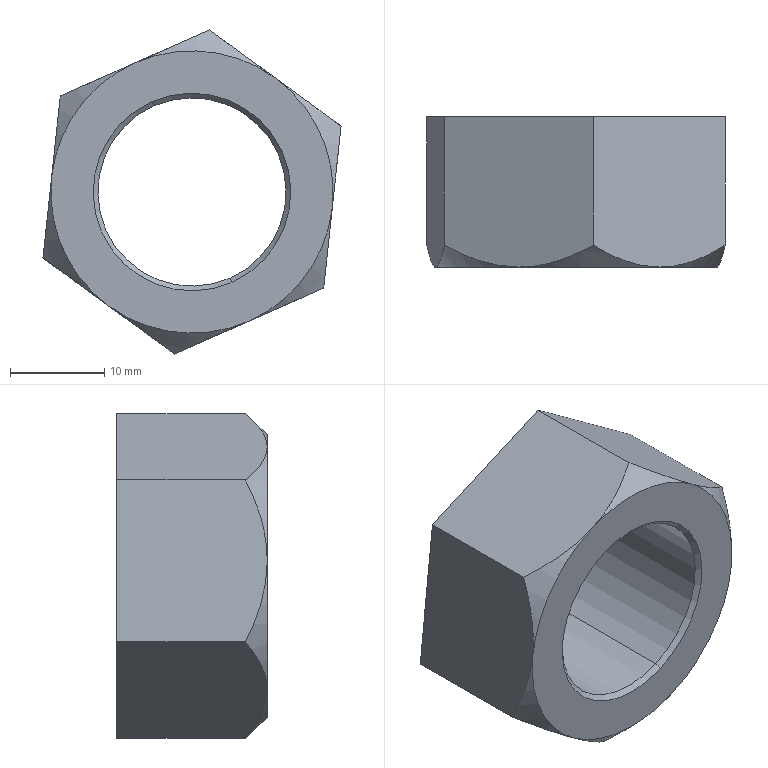Component | SolidWorks | 30-01A-1_Wheel-322-1_FBR100-20-322-1_FBR20nut-322-1 | 1 solid | 20 faces | box 31.68 x 16 x 34.44 mm | volume 7377 mm3 | cone 10 | plane 8 | cylinder 2 | commonest cylinder face diameters 20 x2
STEP:
#1=CARTESIAN_POINT('',(9.316,-22.179,-1.147));
#2=VERTEX_POINT('',#1);
#3=CARTESIAN_POINT('',(8.997,-22.179,-0.4274));
#4=VERTEX_POINT('',#3);
#5=CARTESIAN_POINT('',(9.156,-22.179,-0.7874));
#6=DIRECTION('',(-0.,-1.,0.));
#7=DIRECTION('',(-0.4048,0.,0.9144));
#8=AXIS2_PLACEMENT_3D('',#5,#6,#7);
#9=CIRCLE('',#8,0.3937);
#10=EDGE_CURVE('',#2,#4,#9,.T.);
#11=ORIENTED_EDGE('',*,*,#10,.T.);
#12=CARTESIAN_POINT('',(8.989,-22.159,-0.4094));
#13=VERTEX_POINT('',#12);
#14=CARTESIAN_POINT('',(8.989,-22.159,-0.4094));
#15=DIRECTION('',(-0.2863,0.7071,0.6466));
#16=VECTOR('',#15,39.37);
#17=LINE('',#14,#16);
#18=EDGE_CURVE('',#4,#13,#17,.T.);
#19=ORIENTED_EDGE('',*,*,#18,.T.);
#20=CARTESIAN_POINT('',(9.324,-22.159,-1.165));
#21=VERTEX_POINT('',#20);
#22=CARTESIAN_POINT('',(9.156,-22.159,-0.7874));
#23=DIRECTION('',(-0.,-1.,0.));
#24=DIRECTION('',(-0.4048,0.,0.9144));
#25=AXIS2_PLACEMENT_3D('',#22,#23,#24);
#26=CIRCLE('',#25,0.4134);
#27=EDGE_CURVE('',#21,#13,#26,.T.);
#28=ORIENTED_EDGE('',*,*,#27,.F.);
#29=CARTESIAN_POINT('',(9.324,-22.159,-1.165));
#30=DIRECTION('',(0.2863,0.7071,-0.6466));
#31=VECTOR('',#30,39.37);
#32=LINE('',#29,#31);
#33=EDGE_CURVE('',#2,#21,#32,.T.);
#34=ORIENTED_EDGE('',*,*,#33,.F.);
#35=EDGE_LOOP('',(#11,#19,#28,#34));
#36=FACE_OUTER_BOUND('',#35,.T.);
#37=CARTESIAN_POINT('',(9.156,-22.159,-0.7874));
#38=DIRECTION('',(0.,1.,-0.));
#39=DIRECTION('',(0.4048,0.,-0.9144));
#40=AXIS2_PLACEMENT_3D('',#37,#38,#39);
#41=CONICAL_SURFACE('',#40,0.4134,0.7854);
#42=ADVANCED_FACE('',(#36),#41,.F.);
#43=ORIENTED_EDGE('',*,*,#10,.F.);
#44=CARTESIAN_POINT('',(9.316,-22.769,-1.147));
#45=VERTEX_POINT('',#44);
#46=CARTESIAN_POINT('',(9.316,-22.159,-1.147));
#47=DIRECTION('',(-0.,-1.,0.));
#48=VECTOR('',#47,39.37);
#49=LINE('',#46,#48);
#50=EDGE_CURVE('',#2,#45,#49,.T.);
#51=ORIENTED_EDGE('',*,*,#50,.T.);
#52=CARTESIAN_POINT('',(8.997,-22.769,-0.4274));
#53=VERTEX_POINT('',#52);
#54=CARTESIAN_POINT('',(9.156,-22.769,-0.7874));
#55=DIRECTION('',(-0.,-1.,0.));
#56=DIRECTION('',(-0.4048,0.,0.9144));
#57=AXIS2_PLACEMENT_3D('',#54,#55,#56);
#58=CIRCLE('',#57,0.3937);
#59=EDGE_CURVE('',#45,#53,#58,.T.);
#60=ORIENTED_EDGE('',*,*,#59,.T.);
#61=CARTESIAN_POINT('',(8.997,-22.159,-0.4274));
#62=DIRECTION('',(-0.,-1.,0.));
#63=VECTOR('',#62,39.37);
#64=LINE('',#61,#63);
#65=EDGE_CURVE('',#4,#53,#64,.T.);
#66=ORIENTED_EDGE('',*,*,#65,.F.);
#67=EDGE_LOOP('',(#43,#51,#60,#66));
#68=FACE_OUTER_BOUND('',#67,.T.);
#69=CARTESIAN_POINT('',(9.156,-22.159,-0.7874));
#70=DIRECTION('',(-0.,-1.,0.));
#71=DIRECTION('',(-0.4048,0.,0.9144));
#72=AXIS2_PLACEMENT_3D('',#69,#70,#71);
#73=CYLINDRICAL_SURFACE('',#72,0.3937);
#74=ADVANCED_FACE('',(#68),#73,.F.);
#75=ORIENTED_EDGE('',*,*,#59,.F.);
#76=CARTESIAN_POINT('',(9.324,-22.789,-1.165));
#77=VERTEX_POINT('',#76);
#78=CARTESIAN_POINT('',(9.316,-22.769,-1.147));
#79=DIRECTION('',(0.2863,-0.7071,-0.6466));
#80=VECTOR('',#79,39.37);
#81=LINE('',#78,#80);
#82=EDGE_CURVE('',#45,#77,#81,.T.);
#83=ORIENTED_EDGE('',*,*,#82,.T.);
#84=CARTESIAN_POINT('',(8.989,-22.789,-0.4094));
#85=VERTEX_POINT('',#84);
#86=CARTESIAN_POINT('',(9.156,-22.789,-0.7874));
#87=DIRECTION('',(-0.,-1.,0.));
#88=DIRECTION('',(-0.4048,0.,0.9144));
#89=AXIS2_PLACEMENT_3D('',#86,#87,#88);
#90=CIRCLE('',#89,0.4134);
#91=EDGE_CURVE('',#77,#85,#90,.T.);
#92=ORIENTED_EDGE('',*,*,#91,.T.);
#93=CARTESIAN_POINT('',(8.997,-22.769,-0.4274));
#94=DIRECTION('',(-0.2863,-0.7071,0.6466));
#95=VECTOR('',#94,39.37);
#96=LINE('',#93,#95);
#97=EDGE_CURVE('',#53,#85,#96,.T.);
#98=ORIENTED_EDGE('',*,*,#97,.F.);
#99=EDGE_LOOP('',(#75,#83,#92,#98));
#100=FACE_OUTER_BOUND('',#99,.T.);
#101=CARTESIAN_POINT('',(9.156,-22.769,-0.7874));
#102=DIRECTION('',(-0.,-1.,0.));
#103=DIRECTION('',(-0.4048,0.,0.9144));
#104=AXIS2_PLACEMENT_3D('',#101,#102,#103);
#105=CONICAL_SURFACE('',#104,0.3937,0.7854);
#106=ADVANCED_FACE('',(#100),#105,.F.);
#107=CARTESIAN_POINT('',(8.917,-22.789,-0.2474));
#108=VERTEX_POINT('',#107);
#109=CARTESIAN_POINT('',(8.569,-22.789,-0.7245));
#110=VERTEX_POINT('',#109);
#111=CARTESIAN_POINT('',(9.156,-22.789,-0.7874));
#112=DIRECTION('',(-0.,-1.,0.));
#113=DIRECTION('',(-0.4048,0.,0.9144));
#114=AXIS2_PLACEMENT_3D('',#111,#112,#113);
#115=CIRCLE('',#114,0.5906);
#116=EDGE_CURVE('',#108,#110,#115,.T.);
#117=ORIENTED_EDGE('',*,*,#116,.T.);
#118=CARTESIAN_POINT('',(8.808,-22.789,-1.264));
#119=VERTEX_POINT('',#118);
#120=CARTESIAN_POINT('',(9.156,-22.789,-0.7874));
#121=DIRECTION('',(-0.,-1.,0.));
#122=DIRECTION('',(-0.4048,0.,0.9144));
#123=AXIS2_PLACEMENT_3D('',#120,#121,#122);
#124=CIRCLE('',#123,0.5906);
#125=EDGE_CURVE('',#110,#119,#124,.T.);
#126=ORIENTED_EDGE('',*,*,#125,.T.);
#127=CARTESIAN_POINT('',(9.395,-22.789,-1.327));
#128=VERTEX_POINT('',#127);
#129=CARTESIAN_POINT('',(9.156,-22.789,-0.7874));
#130=DIRECTION('',(-0.,-1.,0.));
#131=DIRECTION('',(-0.4048,0.,0.9144));
#132=AXIS2_PLACEMENT_3D('',#129,#130,#131);
#133=CIRCLE('',#132,0.5906);
#134=EDGE_CURVE('',#119,#128,#133,.T.);
#135=ORIENTED_EDGE('',*,*,#134,.T.);
#136=CARTESIAN_POINT('',(9.743,-22.789,-0.8503));
#137=VERTEX_POINT('',#136);
#138=CARTESIAN_POINT('',(9.156,-22.789,-0.7874));
#139=DIRECTION('',(-0.,-1.,0.));
#140=DIRECTION('',(-0.4048,0.,0.9144));
#141=AXIS2_PLACEMENT_3D('',#138,#139,#140);
#142=CIRCLE('',#141,0.5906);
#143=EDGE_CURVE('',#128,#137,#142,.T.);
#144=ORIENTED_EDGE('',*,*,#143,.T.);
#145=CARTESIAN_POINT('',(9.504,-22.789,-0.3104));
#146=VERTEX_POINT('',#145);
#147=CARTESIAN_POINT('',(9.156,-22.789,-0.7874));
#148=DIRECTION('',(-0.,-1.,0.));
#149=DIRECTION('',(-0.4048,0.,0.9144));
#150=AXIS2_PLACEMENT_3D('',#147,#148,#149);
#151=CIRCLE('',#150,0.5906);
#152=EDGE_CURVE('',#137,#146,#151,.T.);
#153=ORIENTED_EDGE('',*,*,#152,.T.);
#154=CARTESIAN_POINT('',(9.156,-22.789,-0.7874));
#155=DIRECTION('',(-0.,-1.,0.));
#156=DIRECTION('',(-0.4048,0.,0.9144));
#157=AXIS2_PLACEMENT_3D('',#154,#155,#156);
#158=CIRCLE('',#157,0.5906);
#159=EDGE_CURVE('',#146,#108,#158,.T.);
#160=ORIENTED_EDGE('',*,*,#159,.T.);
#161=EDGE_LOOP('',(#117,#126,#135,#144,#153,#160));
#162=FACE_OUTER_BOUND('',#161,.T.);
#163=CARTESIAN_POINT('',(9.156,-22.789,-0.7874));
#164=DIRECTION('',(-0.,-1.,0.));
#165=DIRECTION('',(-0.4048,0.,0.9144));
#166=AXIS2_PLACEMENT_3D('',#163,#164,#165);
#167=CIRCLE('',#166,0.4134);
#168=EDGE_CURVE('',#85,#77,#167,.T.);
#169=ORIENTED_EDGE('',*,*,#168,.F.);
#170=ORIENTED_EDGE('',*,*,#91,.F.);
#171=EDGE_LOOP('',(#169,#170));
#172=FACE_BOUND('',#171,.T.);
#173=CARTESIAN_POINT('',(9.156,-22.789,-0.7874));
#174=DIRECTION('',(0.,1.,-0.));
#175=DIRECTION('',(0.4048,-0.,-0.9144));
#176=AXIS2_PLACEMENT_3D('',#173,#174,#175);
#177=PLANE('',#176);
#178=ADVANCED_FACE('',(#162,#172),#177,.F.);
#179=CARTESIAN_POINT('',(9.78,-22.159,-0.5113));
#180=VERTEX_POINT('',#179);
#181=CARTESIAN_POINT('',(9.229,-22.159,-0.1094));
#182=VERTEX_POINT('',#181);
#183=CARTESIAN_POINT('',(9.78,-22.159,-0.5113));
#184=DIRECTION('',(-0.8078,0.,0.5895));
#185=VECTOR('',#184,39.37);
#186=LINE('',#183,#185);
#187=EDGE_CURVE('',#180,#182,#186,.T.);
#188=ORIENTED_EDGE('',*,*,#187,.F.);
#189=CARTESIAN_POINT('',(9.707,-22.159,-1.189));
#190=VERTEX_POINT('',#189);
#191=CARTESIAN_POINT('',(9.707,-22.159,-1.189));
#192=DIRECTION('',(0.1066,0.,0.9943));
#193=VECTOR('',#192,39.37);
#194=LINE('',#191,#193);
#195=EDGE_CURVE('',#190,#180,#194,.T.);
#196=ORIENTED_EDGE('',*,*,#195,.F.);
#197=CARTESIAN_POINT('',(9.084,-22.159,-1.465));
#198=VERTEX_POINT('',#197);
#199=CARTESIAN_POINT('',(9.084,-22.159,-1.465));
#200=DIRECTION('',(0.9144,-0.,0.4048));
#201=VECTOR('',#200,39.37);
#202=LINE('',#199,#201);
#203=EDGE_CURVE('',#198,#190,#202,.T.);
#204=ORIENTED_EDGE('',*,*,#203,.F.);
#205=CARTESIAN_POINT('',(8.533,-22.159,-1.063));
#206=VERTEX_POINT('',#205);
#207=CARTESIAN_POINT('',(8.533,-22.159,-1.063));
#208=DIRECTION('',(0.8078,-0.,-0.5895));
#209=VECTOR('',#208,39.37);
#210=LINE('',#207,#209);
#211=EDGE_CURVE('',#206,#198,#210,.T.);
#212=ORIENTED_EDGE('',*,*,#211,.F.);
#213=CARTESIAN_POINT('',(8.605,-22.159,-0.3854));
#214=VERTEX_POINT('',#213);
#215=CARTESIAN_POINT('',(8.605,-22.159,-0.3854));
#216=DIRECTION('',(-0.1066,-0.,-0.9943));
#217=VECTOR('',#216,39.37);
#218=LINE('',#215,#217);
#219=EDGE_CURVE('',#214,#206,#218,.T.);
#220=ORIENTED_EDGE('',*,*,#219,.F.);
#221=CARTESIAN_POINT('',(9.229,-22.159,-0.1094));
#222=DIRECTION('',(-0.9144,0.,-0.4048));
#223=VECTOR('',#222,39.37);
#224=LINE('',#221,#223);
#225=EDGE_CURVE('',#182,#214,#224,.T.);
#226=ORIENTED_EDGE('',*,*,#225,.F.);
#227=EDGE_LOOP('',(#188,#196,#204,#212,#220,#226));
#228=FACE_OUTER_BOUND('',#227,.T.);
#229=ORIENTED_EDGE('',*,*,#27,.T.);
#230=CARTESIAN_POINT('',(9.156,-22.159,-0.7874));
#231=DIRECTION('',(-0.,-1.,0.));
#232=DIRECTION('',(-0.4048,0.,0.9144));
#233=AXIS2_PLACEMENT_3D('',#230,#231,#232);
#234=CIRCLE('',#233,0.4134);
#235=EDGE_CURVE('',#13,#21,#234,.T.);
#236=ORIENTED_EDGE('',*,*,#235,.T.);
#237=EDGE_LOOP('',(#229,#236));
#238=FACE_BOUND('',#237,.T.);
#239=CARTESIAN_POINT('',(8.508,-22.159,-1.074));
#240=DIRECTION('',(-0.,-1.,0.));
#241=DIRECTION('',(-0.4048,0.,0.9144));
#242=AXIS2_PLACEMENT_3D('',#239,#240,#241);
#243=PLANE('',#242);
#244=ADVANCED_FACE('',(#228,#238),#243,.F.);
#245=CARTESIAN_POINT('',(9.707,-22.698,-1.189));
#246=VERTEX_POINT('',#245);
#247=CARTESIAN_POINT('',(9.395,-22.789,-1.327));
#248=CARTESIAN_POINT('',(9.409,-22.789,-1.321));
#249=CARTESIAN_POINT('',(9.423,-22.789,-1.315));
#250=CARTESIAN_POINT('',(9.45,-22.786,-1.303));
#251=CARTESIAN_POINT('',(9.463,-22.785,-1.297));
#252=CARTESIAN_POINT('',(9.504,-22.778,-1.279));
#253=CARTESIAN_POINT('',(9.53,-22.772,-1.268));
#254=CARTESIAN_POINT('',(9.582,-22.756,-1.245));
#255=CARTESIAN_POINT('',(9.608,-22.746,-1.233));
#256=CARTESIAN_POINT('',(9.658,-22.723,-1.211));
#257=CARTESIAN_POINT('',(9.683,-22.711,-1.2));
#258=CARTESIAN_POINT('',(9.707,-22.698,-1.189));
#259=B_SPLINE_CURVE_WITH_KNOTS('',3,(#247,#248,#249,#250,#251,#252,#253,#254,#255,#256,#257,#258),.UNSPECIFIED.,.F.,.F.,(4,2,2,2,2,4),(0.01814,0.01926,0.02038,0.02262,0.02486,0.02711),.UNSPECIFIED.);
#260=EDGE_CURVE('',#128,#246,#259,.T.);
#261=ORIENTED_EDGE('',*,*,#260,.T.);
#262=CARTESIAN_POINT('',(9.707,-22.698,-1.189));
#263=CARTESIAN_POINT('',(9.713,-22.725,-1.136));
#264=CARTESIAN_POINT('',(9.719,-22.747,-1.082));
#265=CARTESIAN_POINT('',(9.728,-22.772,-0.9974));
#266=CARTESIAN_POINT('',(9.731,-22.778,-0.9687));
#267=CARTESIAN_POINT('',(9.737,-22.787,-0.9102));
#268=CARTESIAN_POINT('',(9.74,-22.789,-0.88));
#269=CARTESIAN_POINT('',(9.743,-22.789,-0.8503));
#270=B_SPLINE_CURVE_WITH_KNOTS('',3,(#262,#263,#264,#265,#266,#267,#268,#269),.UNSPECIFIED.,.F.,.F.,(4,2,2,4),(0.00000025,0.004489,0.006733,0.008977),.UNSPECIFIED.);
#271=EDGE_CURVE('',#246,#137,#270,.T.);
#272=ORIENTED_EDGE('',*,*,#271,.T.);
#273=ORIENTED_EDGE('',*,*,#143,.F.);
#274=EDGE_LOOP('',(#261,#272,#273));
#275=FACE_OUTER_BOUND('',#274,.T.);
#276=CARTESIAN_POINT('',(9.156,-22.671,-0.7874));
#277=DIRECTION('',(0.,1.,-0.));
#278=DIRECTION('',(0.4048,0.,-0.9144));
#279=AXIS2_PLACEMENT_3D('',#276,#277,#278);
#280=CONICAL_SURFACE('',#279,0.7087,0.7854);
#281=ADVANCED_FACE('',(#275),#280,.T.);
#282=ORIENTED_EDGE('',*,*,#152,.F.);
#283=CARTESIAN_POINT('',(9.78,-22.698,-0.5113));
#284=VERTEX_POINT('',#283);
#285=CARTESIAN_POINT('',(9.743,-22.789,-0.8503));
#286=CARTESIAN_POINT('',(9.75,-22.789,-0.7914));
#287=CARTESIAN_POINT('',(9.756,-22.78,-0.7334));
#288=CARTESIAN_POINT('',(9.768,-22.747,-0.6191));
#289=CARTESIAN_POINT('',(9.774,-22.724,-0.5644));
#290=CARTESIAN_POINT('',(9.78,-22.698,-0.5113));
#291=B_SPLINE_CURVE_WITH_KNOTS('',3,(#285,#286,#287,#288,#289,#290),.UNSPECIFIED.,.F.,.F.,(4,2,4),(0.008977,0.01343,0.01789),.UNSPECIFIED.);
#292=EDGE_CURVE('',#137,#284,#291,.T.);
#293=ORIENTED_EDGE('',*,*,#292,.T.);
#294=CARTESIAN_POINT('',(9.78,-22.698,-0.5113));
#295=CARTESIAN_POINT('',(9.737,-22.725,-0.4798));
#296=CARTESIAN_POINT('',(9.692,-22.747,-0.4476));
#297=CARTESIAN_POINT('',(9.624,-22.772,-0.3975));
#298=CARTESIAN_POINT('',(9.601,-22.778,-0.3805));
#299=CARTESIAN_POINT('',(9.553,-22.787,-0.3458));
#300=CARTESIAN_POINT('',(9.529,-22.789,-0.328));
#301=CARTESIAN_POINT('',(9.504,-22.789,-0.3104));
#302=B_SPLINE_CURVE_WITH_KNOTS('',3,(#294,#295,#296,#297,#298,#299,#300,#301),.UNSPECIFIED.,.F.,.F.,(4,2,2,4),(0.00000025,0.004489,0.006733,0.008977),.UNSPECIFIED.);
#303=EDGE_CURVE('',#284,#146,#302,.T.);
#304=ORIENTED_EDGE('',*,*,#303,.T.);
#305=EDGE_LOOP('',(#282,#293,#304));
#306=FACE_OUTER_BOUND('',#305,.T.);
#307=CARTESIAN_POINT('',(9.156,-22.671,-0.7874));
#308=DIRECTION('',(0.,1.,-0.));
#309=DIRECTION('',(0.4048,0.,-0.9144));
#310=AXIS2_PLACEMENT_3D('',#307,#308,#309);
#311=CONICAL_SURFACE('',#310,0.7087,0.7854);
#312=ADVANCED_FACE('',(#306),#311,.T.);
#313=ORIENTED_EDGE('',*,*,#159,.F.);
#314=CARTESIAN_POINT('',(9.229,-22.698,-0.1094));
#315=VERTEX_POINT('',#314);
#316=CARTESIAN_POINT('',(9.504,-22.789,-0.3104));
#317=CARTESIAN_POINT('',(9.457,-22.789,-0.2754));
#318=CARTESIAN_POINT('',(9.409,-22.78,-0.241));
#319=CARTESIAN_POINT('',(9.317,-22.747,-0.1733));
#320=CARTESIAN_POINT('',(9.272,-22.724,-0.1409));
#321=CARTESIAN_POINT('',(9.229,-22.698,-0.1094));
#322=B_SPLINE_CURVE_WITH_KNOTS('',3,(#316,#317,#318,#319,#320,#321),.UNSPECIFIED.,.F.,.F.,(4,2,4),(0.008977,0.01343,0.01789),.UNSPECIFIED.);
#323=EDGE_CURVE('',#146,#315,#322,.T.);
#324=ORIENTED_EDGE('',*,*,#323,.T.);
#325=CARTESIAN_POINT('',(9.229,-22.698,-0.1094));
#326=CARTESIAN_POINT('',(9.205,-22.711,-0.1201));
#327=CARTESIAN_POINT('',(9.18,-22.723,-0.131));
#328=CARTESIAN_POINT('',(9.129,-22.746,-0.1535));
#329=CARTESIAN_POINT('',(9.104,-22.756,-0.1648));
#330=CARTESIAN_POINT('',(9.052,-22.772,-0.1878));
#331=CARTESIAN_POINT('',(9.025,-22.778,-0.1995));
#332=CARTESIAN_POINT('',(8.985,-22.785,-0.2173));
#333=CARTESIAN_POINT('',(8.972,-22.786,-0.2232));
#334=CARTESIAN_POINT('',(8.945,-22.789,-0.2353));
#335=CARTESIAN_POINT('',(8.931,-22.789,-0.2414));
#336=CARTESIAN_POINT('',(8.917,-22.789,-0.2474));
#337=B_SPLINE_CURVE_WITH_KNOTS('',3,(#325,#326,#327,#328,#329,#330,#331,#332,#333,#334,#335,#336),.UNSPECIFIED.,.F.,.F.,(4,2,2,2,2,4),(0.0116,0.01384,0.01608,0.01833,0.01945,0.02057),.UNSPECIFIED.);
#338=EDGE_CURVE('',#315,#108,#337,.T.);
#339=ORIENTED_EDGE('',*,*,#338,.T.);
#340=EDGE_LOOP('',(#313,#324,#339));
#341=FACE_OUTER_BOUND('',#340,.T.);
#342=CARTESIAN_POINT('',(9.156,-22.671,-0.7874));
#343=DIRECTION('',(0.,1.,-0.));
#344=DIRECTION('',(0.4048,0.,-0.9144));
#345=AXIS2_PLACEMENT_3D('',#342,#343,#344);
#346=CONICAL_SURFACE('',#345,0.7087,0.7854);
#347=ADVANCED_FACE('',(#341),#346,.T.);
#348=ORIENTED_EDGE('',*,*,#116,.F.);
#349=CARTESIAN_POINT('',(8.605,-22.698,-0.3854));
#350=VERTEX_POINT('',#349);
#351=CARTESIAN_POINT('',(8.917,-22.789,-0.2474));
#352=CARTESIAN_POINT('',(8.862,-22.789,-0.2717));
#353=CARTESIAN_POINT('',(8.809,-22.78,-0.2953));
#354=CARTESIAN_POINT('',(8.731,-22.755,-0.33));
#355=CARTESIAN_POINT('',(8.705,-22.746,-0.3415));
#356=CARTESIAN_POINT('',(8.654,-22.723,-0.3639));
#357=CARTESIAN_POINT('',(8.63,-22.711,-0.3748));
#358=CARTESIAN_POINT('',(8.605,-22.698,-0.3854));
#359=B_SPLINE_CURVE_WITH_KNOTS('',3,(#351,#352,#353,#354,#355,#356,#357,#358),.UNSPECIFIED.,.F.,.F.,(4,2,2,4),(0.02057,0.02506,0.02731,0.02956),.UNSPECIFIED.);
#360=EDGE_CURVE('',#108,#350,#359,.T.);
#361=ORIENTED_EDGE('',*,*,#360,.T.);
#362=CARTESIAN_POINT('',(8.605,-22.698,-0.3854));
#363=CARTESIAN_POINT('',(8.6,-22.725,-0.4386));
#364=CARTESIAN_POINT('',(8.594,-22.747,-0.493));
#365=CARTESIAN_POINT('',(8.585,-22.772,-0.5775));
#366=CARTESIAN_POINT('',(8.582,-22.778,-0.6061));
#367=CARTESIAN_POINT('',(8.576,-22.787,-0.6646));
#368=CARTESIAN_POINT('',(8.572,-22.789,-0.6948));
#369=CARTESIAN_POINT('',(8.569,-22.789,-0.7245));
#370=B_SPLINE_CURVE_WITH_KNOTS('',3,(#362,#363,#364,#365,#366,#367,#368,#369),.UNSPECIFIED.,.F.,.F.,(4,2,2,4),(0.00000025,0.004489,0.006733,0.008977),.UNSPECIFIED.);
#371=EDGE_CURVE('',#350,#110,#370,.T.);
#372=ORIENTED_EDGE('',*,*,#371,.T.);
#373=EDGE_LOOP('',(#348,#361,#372));
#374=FACE_OUTER_BOUND('',#373,.T.);
#375=CARTESIAN_POINT('',(9.156,-22.671,-0.7874));
#376=DIRECTION('',(0.,1.,-0.));
#377=DIRECTION('',(0.4048,0.,-0.9144));
#378=AXIS2_PLACEMENT_3D('',#375,#376,#377);
#379=CONICAL_SURFACE('',#378,0.7087,0.7854);
#380=ADVANCED_FACE('',(#374),#379,.T.);
#381=ORIENTED_EDGE('',*,*,#125,.F.);
#382=CARTESIAN_POINT('',(8.533,-22.698,-1.063));
#383=VERTEX_POINT('',#382);
#384=CARTESIAN_POINT('',(8.569,-22.789,-0.7245));
#385=CARTESIAN_POINT('',(8.563,-22.789,-0.7834));
#386=CARTESIAN_POINT('',(8.557,-22.78,-0.8414));
#387=CARTESIAN_POINT('',(8.544,-22.747,-0.9557));
#388=CARTESIAN_POINT('',(8.538,-22.724,-1.01));
#389=CARTESIAN_POINT('',(8.533,-22.698,-1.063));
#390=B_SPLINE_CURVE_WITH_KNOTS('',3,(#384,#385,#386,#387,#388,#389),.UNSPECIFIED.,.F.,.F.,(4,2,4),(0.008977,0.01343,0.01789),.UNSPECIFIED.);
#391=EDGE_CURVE('',#110,#383,#390,.T.);
#392=ORIENTED_EDGE('',*,*,#391,.T.);
#393=CARTESIAN_POINT('',(8.533,-22.698,-1.063));
#394=CARTESIAN_POINT('',(8.576,-22.725,-1.095));
#395=CARTESIAN_POINT('',(8.62,-22.747,-1.127));
#396=CARTESIAN_POINT('',(8.689,-22.772,-1.177));
#397=CARTESIAN_POINT('',(8.712,-22.778,-1.194));
#398=CARTESIAN_POINT('',(8.76,-22.787,-1.229));
#399=CARTESIAN_POINT('',(8.784,-22.789,-1.247));
#400=CARTESIAN_POINT('',(8.808,-22.789,-1.264));
#401=B_SPLINE_CURVE_WITH_KNOTS('',3,(#393,#394,#395,#396,#397,#398,#399,#400),.UNSPECIFIED.,.F.,.F.,(4,2,2,4),(0.00000025,0.004489,0.006733,0.008977),.UNSPECIFIED.);
#402=EDGE_CURVE('',#383,#119,#401,.T.);
#403=ORIENTED_EDGE('',*,*,#402,.T.);
#404=EDGE_LOOP('',(#381,#392,#403));
#405=FACE_OUTER_BOUND('',#404,.T.);
#406=CARTESIAN_POINT('',(9.156,-22.671,-0.7874));
#407=DIRECTION('',(0.,1.,-0.));
#408=DIRECTION('',(0.4048,0.,-0.9144));
#409=AXIS2_PLACEMENT_3D('',#406,#407,#408);
#410=CONICAL_SURFACE('',#409,0.7087,0.7854);
#411=ADVANCED_FACE('',(#405),#410,.T.);
#412=ORIENTED_EDGE('',*,*,#134,.F.);
#413=CARTESIAN_POINT('',(9.084,-22.698,-1.465));
#414=VERTEX_POINT('',#413);
#415=CARTESIAN_POINT('',(8.808,-22.789,-1.264));
#416=CARTESIAN_POINT('',(8.856,-22.789,-1.299));
#417=CARTESIAN_POINT('',(8.903,-22.78,-1.334));
#418=CARTESIAN_POINT('',(8.996,-22.747,-1.402));
#419=CARTESIAN_POINT('',(9.04,-22.724,-1.434));
#420=CARTESIAN_POINT('',(9.084,-22.698,-1.465));
#421=B_SPLINE_CURVE_WITH_KNOTS('',3,(#415,#416,#417,#418,#419,#420),.UNSPECIFIED.,.F.,.F.,(4,2,4),(0.008977,0.01343,0.01789),.UNSPECIFIED.);
#422=EDGE_CURVE('',#119,#414,#421,.T.);
#423=ORIENTED_EDGE('',*,*,#422,.T.);
#424=CARTESIAN_POINT('',(9.084,-22.698,-1.465));
#425=CARTESIAN_POINT('',(9.108,-22.711,-1.455));
#426=CARTESIAN_POINT('',(9.132,-22.723,-1.444));
#427=CARTESIAN_POINT('',(9.183,-22.746,-1.422));
#428=CARTESIAN_POINT('',(9.209,-22.755,-1.41));
#429=CARTESIAN_POINT('',(9.287,-22.78,-1.375));
#430=CARTESIAN_POINT('',(9.341,-22.789,-1.352));
#431=CARTESIAN_POINT('',(9.395,-22.789,-1.327));
#432=B_SPLINE_CURVE_WITH_KNOTS('',3,(#424,#425,#426,#427,#428,#429,#430,#431),.UNSPECIFIED.,.F.,.F.,(4,2,2,4),(0.00916,0.0114,0.01365,0.01814),.UNSPECIFIED.);
#433=EDGE_CURVE('',#414,#128,#432,.T.);
#434=ORIENTED_EDGE('',*,*,#433,.T.);
#435=EDGE_LOOP('',(#412,#423,#434));
#436=FACE_OUTER_BOUND('',#435,.T.);
#437=CARTESIAN_POINT('',(9.156,-22.671,-0.7874));
#438=DIRECTION('',(0.,1.,-0.));
#439=DIRECTION('',(0.4048,0.,-0.9144));
#440=AXIS2_PLACEMENT_3D('',#437,#438,#439);
#441=CONICAL_SURFACE('',#440,0.7087,0.7854);
#442=ADVANCED_FACE('',(#436),#441,.T.);
#443=CARTESIAN_POINT('',(9.707,-22.829,-1.189));
#444=DIRECTION('',(0.,1.,-0.));
#445=VECTOR('',#444,39.37);
#446=LINE('',#443,#445);
#447=EDGE_CURVE('',#246,#190,#446,.T.);
#448=ORIENTED_EDGE('',*,*,#447,.T.);
#449=ORIENTED_EDGE('',*,*,#195,.T.);
#450=CARTESIAN_POINT('',(9.78,-22.829,-0.5113));
#451=DIRECTION('',(0.,1.,-0.));
#452=VECTOR('',#451,39.37);
#453=LINE('',#450,#452);
#454=EDGE_CURVE('',#284,#180,#453,.T.);
#455=ORIENTED_EDGE('',*,*,#454,.F.);
#456=ORIENTED_EDGE('',*,*,#292,.F.);
#457=ORIENTED_EDGE('',*,*,#271,.F.);
#458=EDGE_LOOP('',(#448,#449,#455,#456,#457));
#459=FACE_OUTER_BOUND('',#458,.T.);
#460=CARTESIAN_POINT('',(9.707,-22.829,-1.189));
#461=DIRECTION('',(-0.9943,0.,0.1066));
#462=DIRECTION('',(-0.1066,-0.,-0.9943));
#463=AXIS2_PLACEMENT_3D('',#460,#461,#462);
#464=PLANE('',#463);
#465=ADVANCED_FACE('',(#459),#464,.F.);
#466=ORIENTED_EDGE('',*,*,#454,.T.);
#467=ORIENTED_EDGE('',*,*,#187,.T.);
#468=CARTESIAN_POINT('',(9.229,-22.829,-0.1094));
#469=DIRECTION('',(0.,1.,-0.));
#470=VECTOR('',#469,39.37);
#471=LINE('',#468,#470);
#472=EDGE_CURVE('',#315,#182,#471,.T.);
#473=ORIENTED_EDGE('',*,*,#472,.F.);
#474=ORIENTED_EDGE('',*,*,#323,.F.);
#475=ORIENTED_EDGE('',*,*,#303,.F.);
#476=EDGE_LOOP('',(#466,#467,#473,#474,#475));
#477=FACE_OUTER_BOUND('',#476,.T.);
#478=CARTESIAN_POINT('',(9.78,-22.829,-0.5113));
#479=DIRECTION('',(-0.5895,0.,-0.8078));
#480=DIRECTION('',(0.8078,-0.,-0.5895));
#481=AXIS2_PLACEMENT_3D('',#478,#479,#480);
#482=PLANE('',#481);
#483=ADVANCED_FACE('',(#477),#482,.F.);
#484=ORIENTED_EDGE('',*,*,#472,.T.);
#485=ORIENTED_EDGE('',*,*,#225,.T.);
#486=CARTESIAN_POINT('',(8.605,-22.829,-0.3854));
#487=DIRECTION('',(0.,1.,-0.));
#488=VECTOR('',#487,39.37);
#489=LINE('',#486,#488);
#490=EDGE_CURVE('',#350,#214,#489,.T.);
#491=ORIENTED_EDGE('',*,*,#490,.F.);
#492=ORIENTED_EDGE('',*,*,#360,.F.);
#493=ORIENTED_EDGE('',*,*,#338,.F.);
#494=EDGE_LOOP('',(#484,#485,#491,#492,#493));
#495=FACE_OUTER_BOUND('',#494,.T.);
#496=CARTESIAN_POINT('',(9.229,-22.829,-0.1094));
#497=DIRECTION('',(0.4048,-0.,-0.9144));
#498=DIRECTION('',(0.9144,-0.,0.4048));
#499=AXIS2_PLACEMENT_3D('',#496,#497,#498);
#500=PLANE('',#499);
#501=ADVANCED_FACE('',(#495),#500,.F.);
#502=ORIENTED_EDGE('',*,*,#490,.T.);
#503=ORIENTED_EDGE('',*,*,#219,.T.);
#504=CARTESIAN_POINT('',(8.533,-22.829,-1.063));
#505=DIRECTION('',(0.,1.,-0.));
#506=VECTOR('',#505,39.37);
#507=LINE('',#504,#506);
#508=EDGE_CURVE('',#383,#206,#507,.T.);
#509=ORIENTED_EDGE('',*,*,#508,.F.);
#510=ORIENTED_EDGE('',*,*,#391,.F.);
#511=ORIENTED_EDGE('',*,*,#371,.F.);
#512=EDGE_LOOP('',(#502,#503,#509,#510,#511));
#513=FACE_OUTER_BOUND('',#512,.T.);
#514=CARTESIAN_POINT('',(8.605,-22.829,-0.3854));
#515=DIRECTION('',(0.9943,-0.,-0.1066));
#516=DIRECTION('',(0.1066,0.,0.9943));
#517=AXIS2_PLACEMENT_3D('',#514,#515,#516);
#518=PLANE('',#517);
#519=ADVANCED_FACE('',(#513),#518,.F.);
#520=ORIENTED_EDGE('',*,*,#508,.T.);
#521=ORIENTED_EDGE('',*,*,#211,.T.);
#522=CARTESIAN_POINT('',(9.084,-22.829,-1.465));
#523=DIRECTION('',(0.,1.,-0.));
#524=VECTOR('',#523,39.37);
#525=LINE('',#522,#524);
#526=EDGE_CURVE('',#414,#198,#525,.T.);
#527=ORIENTED_EDGE('',*,*,#526,.F.);
#528=ORIENTED_EDGE('',*,*,#422,.F.);
#529=ORIENTED_EDGE('',*,*,#402,.F.);
#530=EDGE_LOOP('',(#520,#521,#527,#528,#529));
#531=FACE_OUTER_BOUND('',#530,.T.);
#532=CARTESIAN_POINT('',(8.533,-22.829,-1.063));
#533=DIRECTION('',(0.5895,-0.,0.8078));
#534=DIRECTION('',(-0.8078,0.,0.5895));
#535=AXIS2_PLACEMENT_3D('',#532,#533,#534);
#536=PLANE('',#535);
#537=ADVANCED_FACE('',(#531),#536,.F.);
#538=ORIENTED_EDGE('',*,*,#526,.T.);
#539=ORIENTED_EDGE('',*,*,#203,.T.);
#540=ORIENTED_EDGE('',*,*,#447,.F.);
#541=ORIENTED_EDGE('',*,*,#260,.F.);
#542=ORIENTED_EDGE('',*,*,#433,.F.);
#543=EDGE_LOOP('',(#538,#539,#540,#541,#542));
#544=FACE_OUTER_BOUND('',#543,.T.);
#545=CARTESIAN_POINT('',(9.084,-22.829,-1.465));
#546=DIRECTION('',(-0.4048,0.,0.9144));
#547=DIRECTION('',(-0.9144,0.,-0.4048));
#548=AXIS2_PLACEMENT_3D('',#545,#546,#547);
#549=PLANE('',#548);
#550=ADVANCED_FACE('',(#544),#549,.F.);
#551=ORIENTED_EDGE('',*,*,#82,.F.);
#552=CARTESIAN_POINT('',(9.156,-22.769,-0.7874));
#553=DIRECTION('',(-0.,-1.,0.));
#554=DIRECTION('',(-0.4048,0.,0.9144));
#555=AXIS2_PLACEMENT_3D('',#552,#553,#554);
#556=CIRCLE('',#555,0.3937);
#557=EDGE_CURVE('',#53,#45,#556,.T.);
#558=ORIENTED_EDGE('',*,*,#557,.F.);
#559=ORIENTED_EDGE('',*,*,#97,.T.);
#560=ORIENTED_EDGE('',*,*,#168,.T.);
#561=EDGE_LOOP('',(#551,#558,#559,#560));
#562=FACE_OUTER_BOUND('',#561,.T.);
#563=CARTESIAN_POINT('',(9.156,-22.769,-0.7874));
#564=DIRECTION('',(-0.,-1.,0.));
#565=DIRECTION('',(-0.4048,0.,0.9144));
#566=AXIS2_PLACEMENT_3D('',#563,#564,#565);
#567=CONICAL_SURFACE('',#566,0.3937,0.7854);
#568=ADVANCED_FACE('',(#562),#567,.F.);
#569=ORIENTED_EDGE('',*,*,#50,.F.);
#570=CARTESIAN_POINT('',(9.156,-22.179,-0.7874));
#571=DIRECTION('',(-0.,-1.,0.));
#572=DIRECTION('',(-0.4048,0.,0.9144));
#573=AXIS2_PLACEMENT_3D('',#570,#571,#572);
#574=CIRCLE('',#573,0.3937);
#575=EDGE_CURVE('',#4,#2,#574,.T.);
#576=ORIENTED_EDGE('',*,*,#575,.F.);
#577=ORIENTED_EDGE('',*,*,#65,.T.);
#578=ORIENTED_EDGE('',*,*,#557,.T.);
#579=EDGE_LOOP('',(#569,#576,#577,#578));
#580=FACE_OUTER_BOUND('',#579,.T.);
#581=CARTESIAN_POINT('',(9.156,-22.159,-0.7874));
#582=DIRECTION('',(-0.,-1.,0.));
#583=DIRECTION('',(-0.4048,0.,0.9144));
#584=AXIS2_PLACEMENT_3D('',#581,#582,#583);
#585=CYLINDRICAL_SURFACE('',#584,0.3937);
#586=ADVANCED_FACE('',(#580),#585,.F.);
#587=ORIENTED_EDGE('',*,*,#18,.F.);
#588=ORIENTED_EDGE('',*,*,#575,.T.);
#589=ORIENTED_EDGE('',*,*,#33,.T.);
#590=ORIENTED_EDGE('',*,*,#235,.F.);
#591=EDGE_LOOP('',(#587,#588,#589,#590));
#592=FACE_OUTER_BOUND('',#591,.T.);
#593=CARTESIAN_POINT('',(9.156,-22.159,-0.7874));
#594=DIRECTION('',(0.,1.,-0.));
#595=DIRECTION('',(0.4048,0.,-0.9144));
#596=AXIS2_PLACEMENT_3D('',#593,#594,#595);
#597=CONICAL_SURFACE('',#596,0.4134,0.7854);
#598=ADVANCED_FACE('',(#592),#597,.F.);
#599=CLOSED_SHELL('',(#42,#74,#106,#178,#244,#281,#312,#347,#380,#411,#442,#465,#483,#501,#519,#537,#550,#568,#586,#598));
#600=MANIFOLD_SOLID_BREP('',#599);
#601=CARTESIAN_POINT('',(0.,0.,0.));
#602=DIRECTION('',(0.,0.,1.));
#603=DIRECTION('',(1.,0.,0.));
#604=AXIS2_PLACEMENT_3D('',#601,#602,#603);
#605=(LENGTH_UNIT()NAMED_UNIT(*)SI_UNIT($,.METRE.));
#606=LENGTH_MEASURE_WITH_UNIT(LENGTH_MEASURE(0.0254),#605);
#607=DIMENSIONAL_EXPONENTS(1.,0.,0.,0.,0.,0.,0.);
#608=(CONVERSION_BASED_UNIT('',#606)LENGTH_UNIT()NAMED_UNIT(#607));
#609=UNCERTAINTY_MEASURE_WITH_UNIT(LENGTH_MEASURE(0.00001),#608,'','');
#610=(NAMED_UNIT(*)PLANE_ANGLE_UNIT()SI_UNIT($,.RADIAN.));
#611=(NAMED_UNIT(*)SI_UNIT($,.STERADIAN.)SOLID_ANGLE_UNIT());
#612=(GEOMETRIC_REPRESENTATION_CONTEXT(3)GLOBAL_UNCERTAINTY_ASSIGNED_CONTEXT((#609))GLOBAL_UNIT_ASSIGNED_CONTEXT((#608,#610,#611))REPRESENTATION_CONTEXT('',''));
#613=ADVANCED_BREP_SHAPE_REPRESENTATION('',(#600,#604),#612);
#614=COLOUR_RGB('',0.7922,0.8196,0.9333);
#615=FILL_AREA_STYLE_COLOUR('',#614);
#616=FILL_AREA_STYLE('',(#615));
#617=SURFACE_STYLE_FILL_AREA(#616);
#618=SURFACE_SIDE_STYLE('',(#617));
#619=SURFACE_STYLE_USAGE(.BOTH.,#618);
#620=PRESENTATION_STYLE_ASSIGNMENT((#619));
#621=STYLED_ITEM('',(#620),#600);
#622=(LENGTH_UNIT()NAMED_UNIT(*)SI_UNIT($,.METRE.));
#623=LENGTH_MEASURE_WITH_UNIT(LENGTH_MEASURE(0.0254),#622);
#624=DIMENSIONAL_EXPONENTS(1.,0.,0.,0.,0.,0.,0.);
#625=(CONVERSION_BASED_UNIT('',#623)LENGTH_UNIT()NAMED_UNIT(#624));
#626=UNCERTAINTY_MEASURE_WITH_UNIT(LENGTH_MEASURE(0.00001),#625,'','');
#627=(NAMED_UNIT(*)PLANE_ANGLE_UNIT()SI_UNIT($,.RADIAN.));
#628=(NAMED_UNIT(*)SI_UNIT($,.STERADIAN.)SOLID_ANGLE_UNIT());
#629=(GEOMETRIC_REPRESENTATION_CONTEXT(3)GLOBAL_UNCERTAINTY_ASSIGNED_CONTEXT((#626))GLOBAL_UNIT_ASSIGNED_CONTEXT((#625,#627,#628))REPRESENTATION_CONTEXT('',''));
#630=MECHANICAL_DESIGN_GEOMETRIC_PRESENTATION_REPRESENTATION('',(#621),#629);
#631=PRESENTATION_LAYER_ASSIGNMENT('','',(#621));